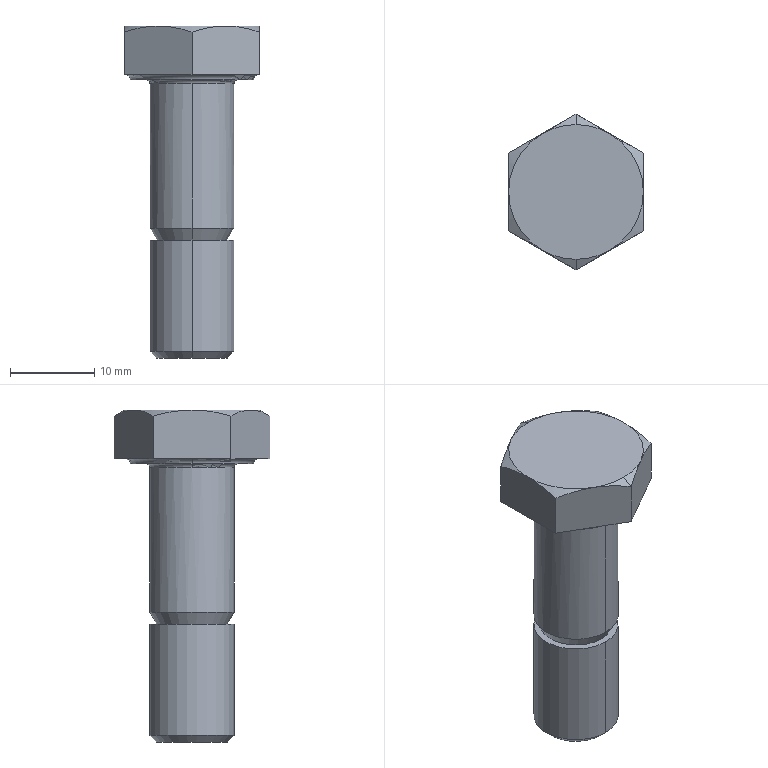Component | NX | BOLT_M10X33_2 | 1 solid | 31 faces | volume 3952 mm3 | cone 12 | plane 11 | cylinder 4 | torus 4 | commonest cylinder face diameters 10 x4